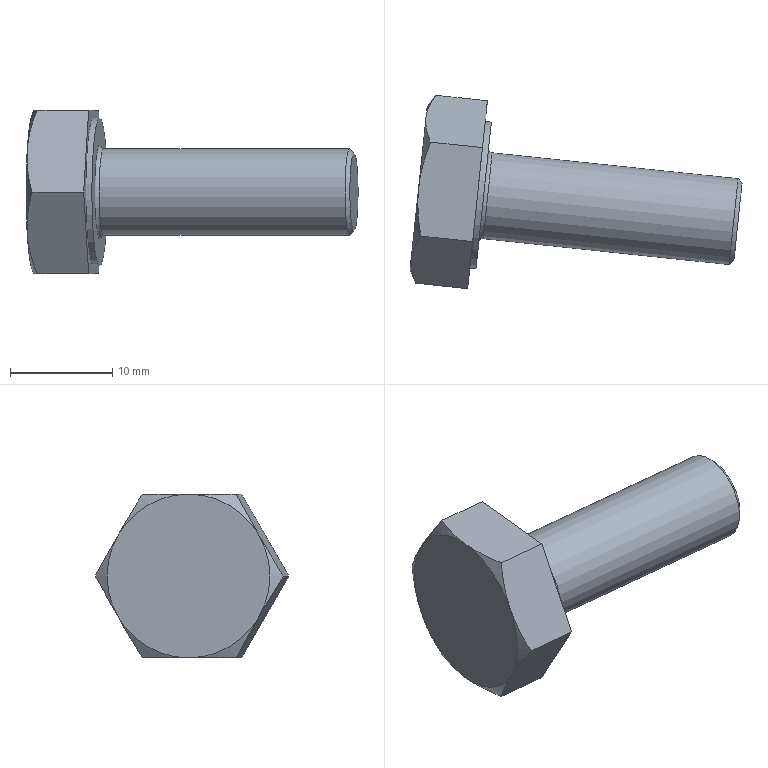Component | NX | GB-T5782-2000_M10X25_3 | 1 solid | 20 faces | volume 2797 mm3 | plane 10 | cone 7 | cylinder 2 | torus 1 | commonest cylinder face diameters 14.47 x1 8.5 x1